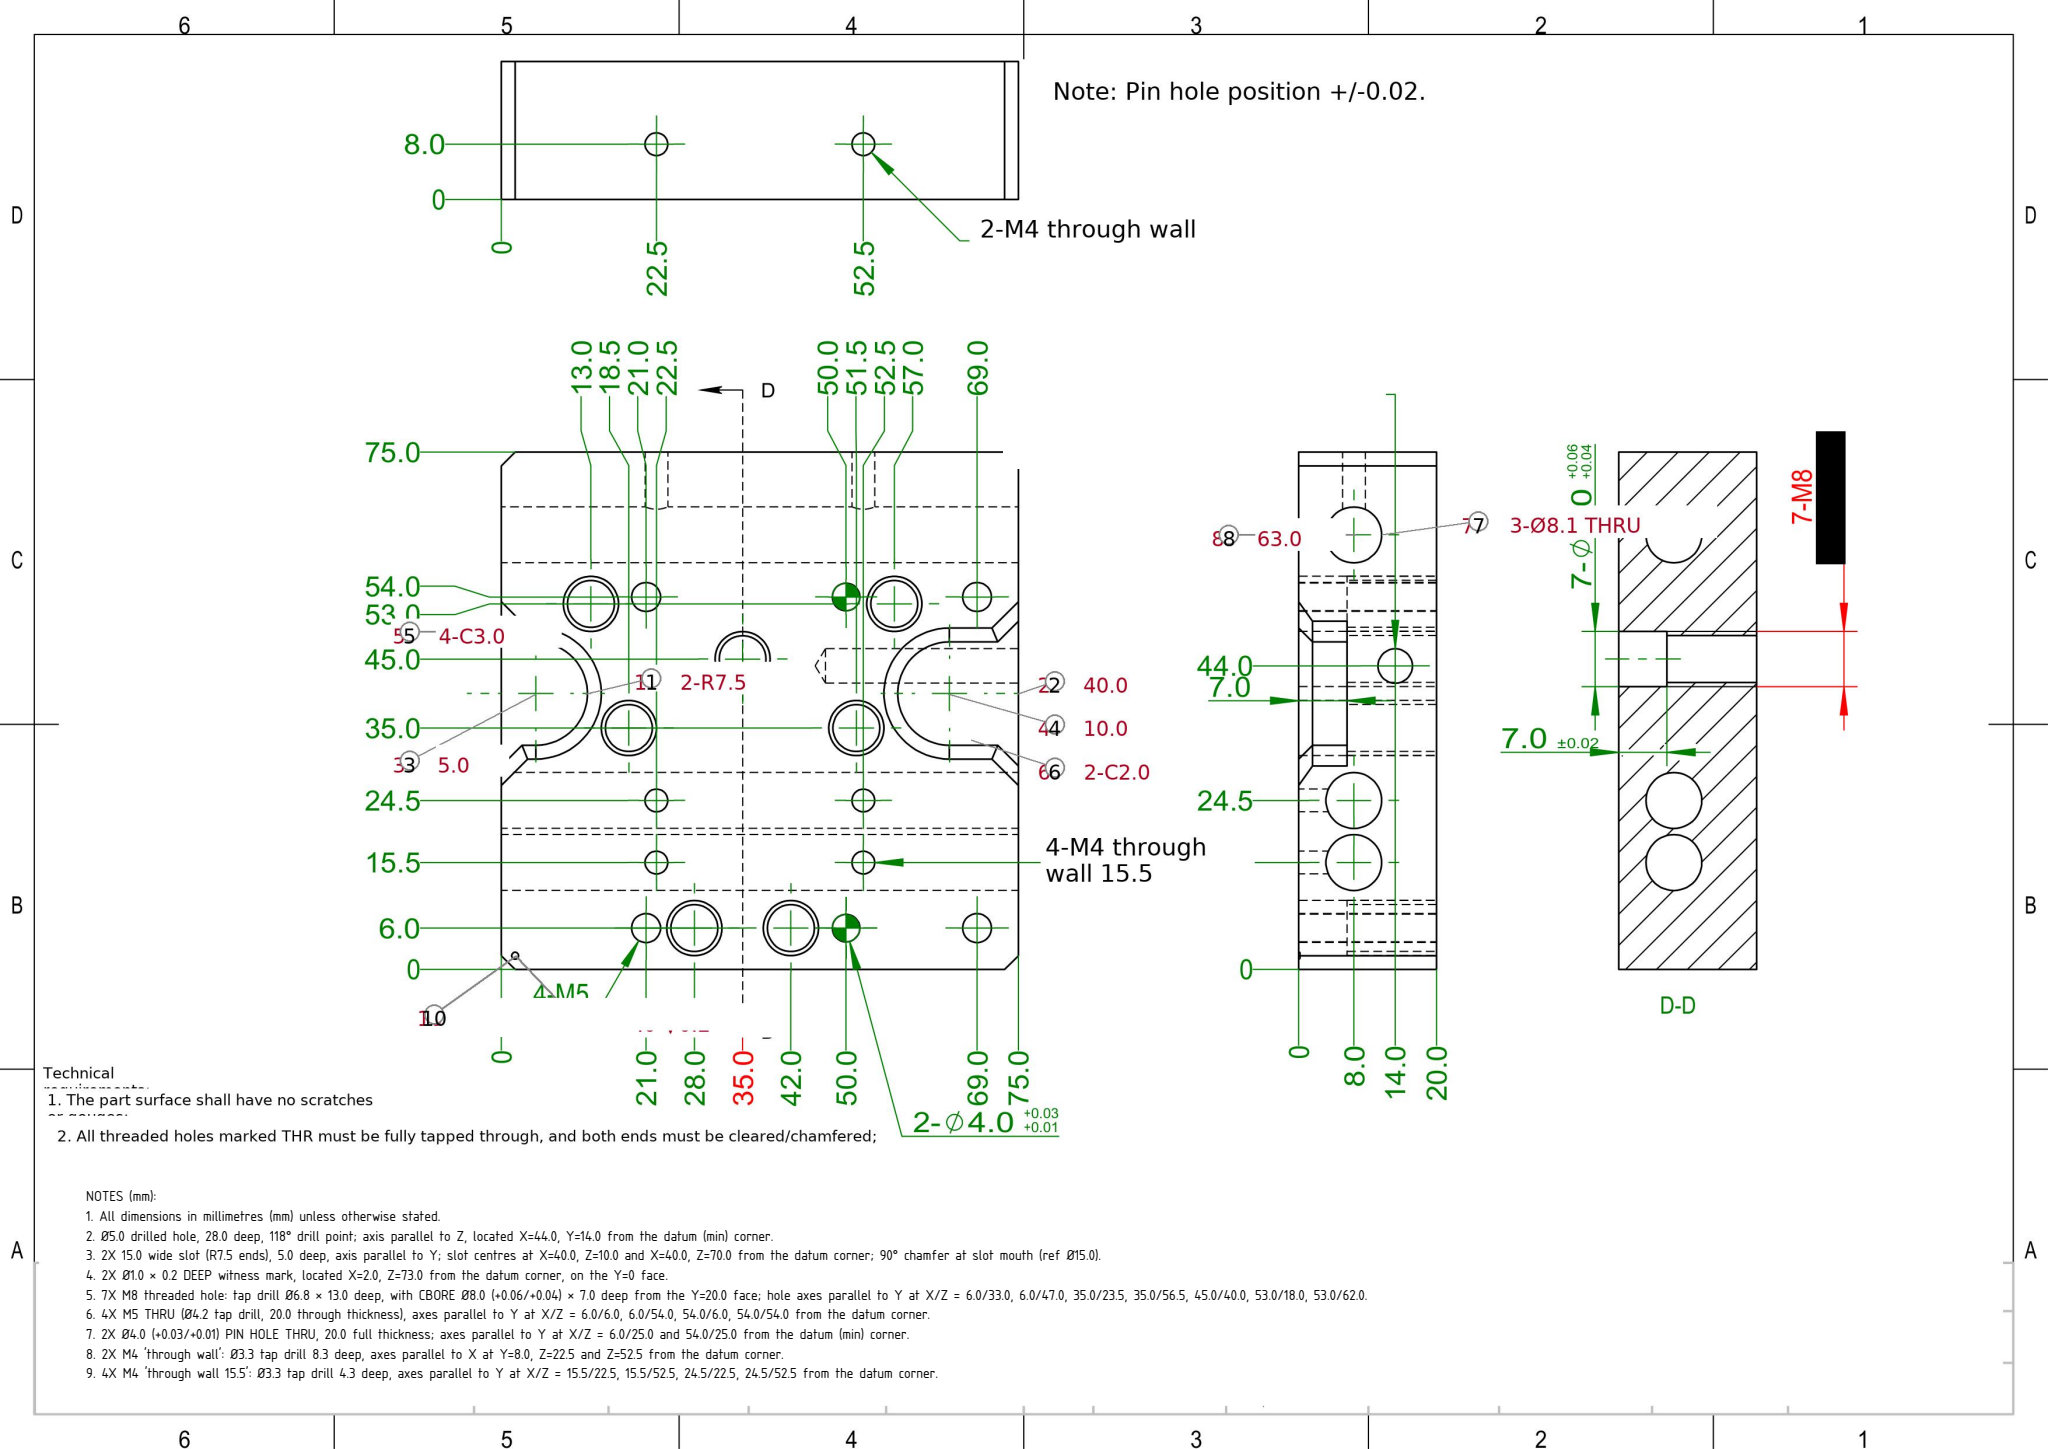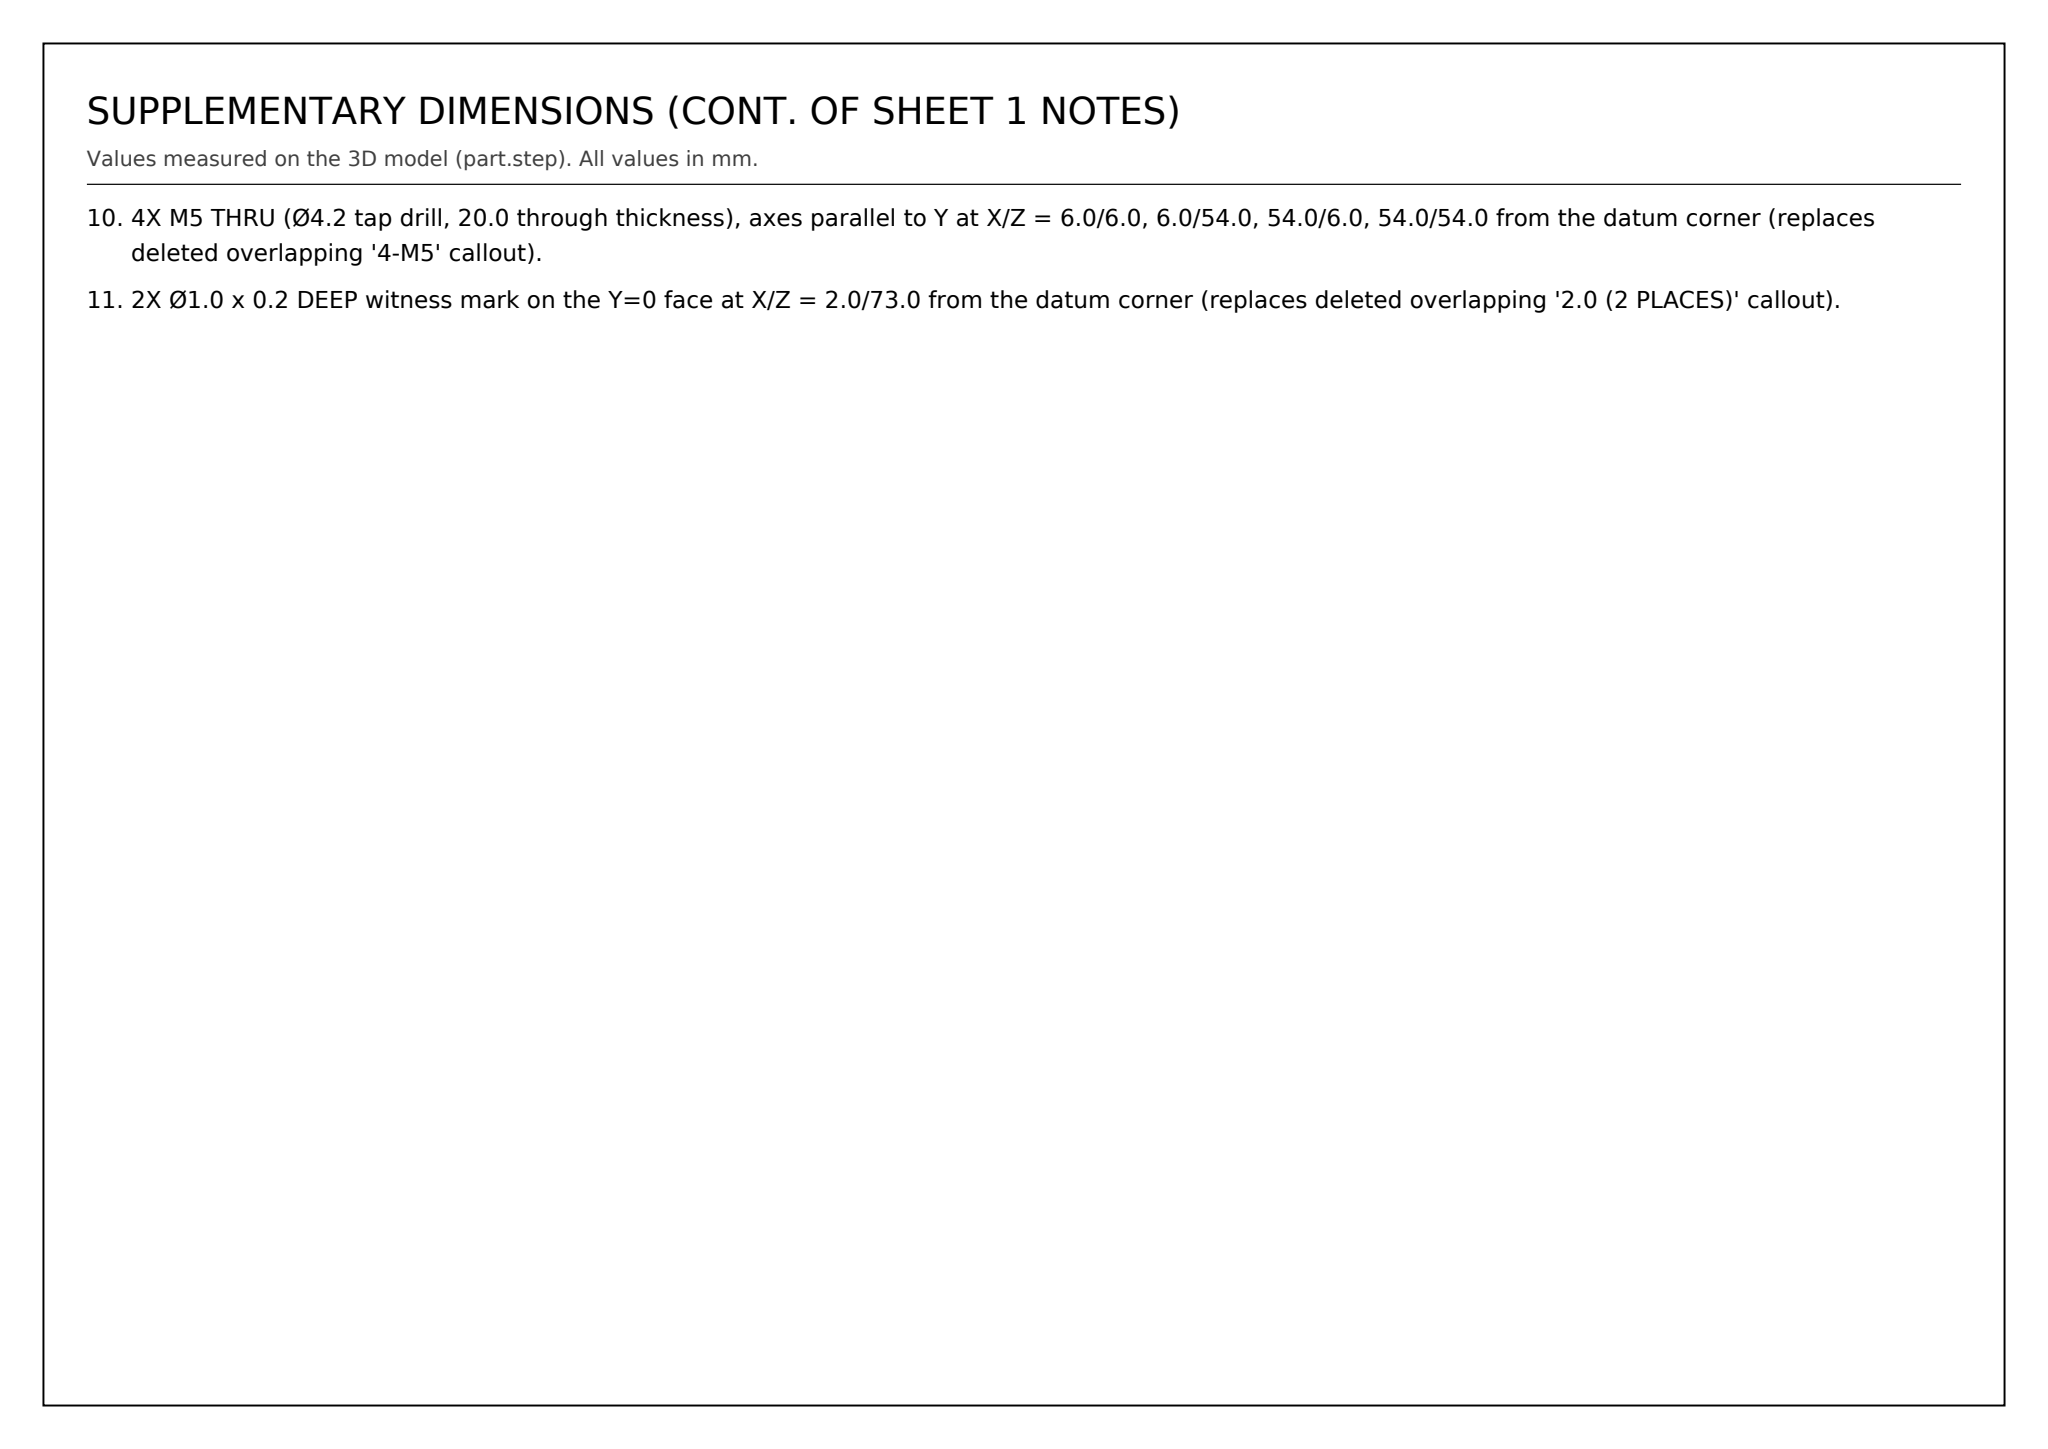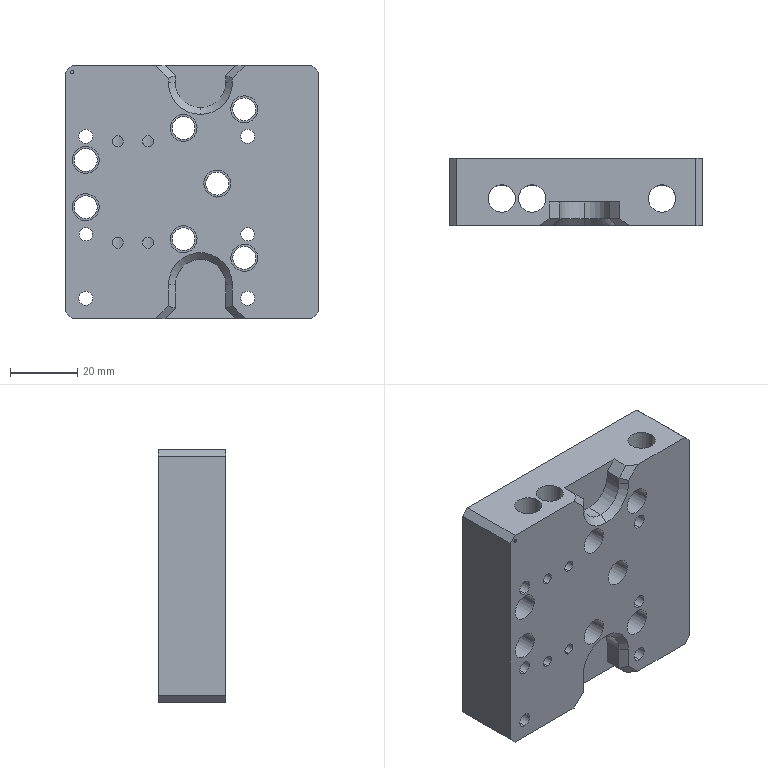Part | SolidWorks | mm | 1 solid | 106 faces | box 75 x 20 x 75 mm | volume 89420 mm3 | cylinder 65 | plane 36 | cone 5 | commonest cylinder face diameters 6.8 x14 8 x14 3.3 x12 4.2 x8 8.1 x6 4 x4 15 x3 1 x2
Drawing notes:
All dimensions in millimetres (mm) unless otherwise stated. | from the solid: STEP model facts header: units mm
Ø5.0 drilled hole, 28.0 deep, 118° drill point; axis parallel to Z, located X=44.0, Y=14.0 from the datum (min) corner. | from the solid: cylinders [5.0,'z',[44.0,14.0],28.0]; cones [118.0, ref dia 5.0]
2X 15.0 wide slot (R7.5 ends), 5.0 deep, axis parallel to Y; slot centres at X=40.0, Z=10.0 and X=40.0, Z=70.0 from the datum corner; 90° chamfer at slot mouth (ref Ø15.0). | from the solid: cylinders [15.0,'y',[40.0,10.0],5.0] and [15.0,'y',[40.0,70.0],5.0]; cones [90.0, ref dia 15.0]
2X Ø1.0 × 0.2 DEEP witness mark, located X=2.0, Z=73.0 from the datum corner, on the Y=0 face. | from the solid: cylinders [1.0,'y',[2.0,73.0],0.2]; axis_planes y 0.0 and y 0.2
7X M8 threaded hole: tap drill Ø6.8 × 13.0 deep, with CBORE Ø8.0 (+0.06/+0.04) × 7.0 deep from the Y=20.0 face; hole axes parallel to Y at X/Z = 6.0/33.0, 6.0/47.0, 35.0/23.5, 35.0/56.5, 45.0/40.0, 53.0/18.0, 53.0/62.0. | from the solid: cylinders [6.8,'y',...,13.0] ×7 and [8.0,'y',same X/Z,7.0] ×7; axis_planes y 7.0 (9), y 20.0
4X M5 THRU (Ø4.2 tap drill, 20.0 through thickness), axes parallel to Y at X/Z = 6.0/6.0, 6.0/54.0, 54.0/6.0, 54.0/54.0 from the datum corner. | from the solid: cylinders [4.2,'y',[6.0,6.0]/[6.0,54.0]/[54.0,6.0]/[54.0,54.0],20.0]
2X Ø4.0 (+0.03/+0.01) PIN HOLE THRU, 20.0 full thickness; axes parallel to Y at X/Z = 6.0/25.0 and 54.0/25.0 from the datum (min) corner. | from the solid: cylinders [4.0,'y',[6.0,null,25.0],20.0] and [4.0,'y',[54.0,null,25.0],20.0]; bbox Y = 20.0
2X M4 'through wall': Ø3.3 tap drill 8.3 deep, axes parallel to X at Y=8.0, Z=22.5 and Z=52.5 from the datum corner. | from the solid: cylinders [3.3,'x',[null,8.0,22.5],8.3,2] and [3.3,'x',[null,8.0,52.5],8.3,2]
4X M4 'through wall 15.5': Ø3.3 tap drill 4.3 deep, axes parallel to Y at X/Z = 15.5/22.5, 15.5/52.5, 24.5/22.5, 24.5/52.5 from the datum corner. | from the solid: cylinders [3.3,'y',[15.5,null,22.5],4.3], [3.3,'y',[15.5,null,52.5],4.3], [3.3,'y',[24.5,null,22.5],4.3], [3.3,'y',[24.5,null,52.5],4.3]
4X M5 THRU (Ø4.2 tap drill, 20.0 through thickness), axes parallel to Y at X/Z = 6.0/6.0, 6.0/54.0, 54.0/6.0, 54.0/54.0 from the datum corner (replaces deleted overlapping '4-M5' callout). | from the solid: cylinders [4.2,'y',[6.0,null,6.0],20.0], [4.2,'y',[6.0,null,54.0],20.0], [4.2,'y',[54.0,null,6.0],20.0], [4.2,'y',[54.0,null,54.0],20.0]
2X Ø1.0 x 0.2 DEEP witness mark on the Y=0 face at X/Z = 2.0/73.0 from the datum corner (replaces deleted overlapping '2.0 (2 PLACES)' callout). | from the solid: cylinders [1.0,'y',[2.0,null,73.0],0.2,2]; plane y=0.2